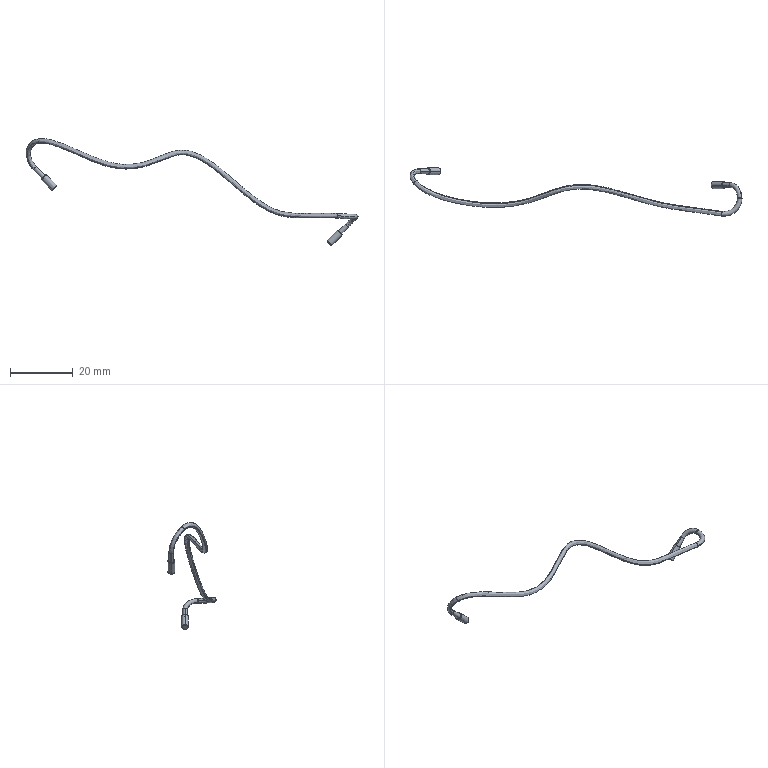Component | SolidWorks | Crijevo_paX2-1 | 3 solids | 56 faces | box 106.11 x 15.45 x 34.2 mm | volume 97 mm3 | cylinder 20 | torus 16 | spline 8 | plane 8 | cone 4 | commonest cylinder face diameters 1.5 x10 1.3 x6 2.2 x4